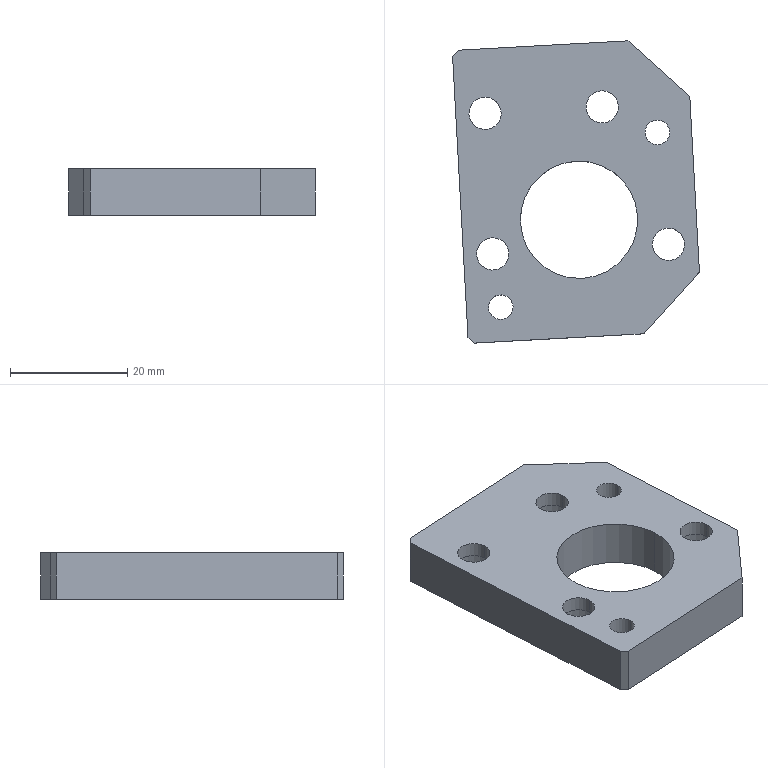Component | SolidWorks | T160418-M01U03-P13A-1 | 1 solid | 36 faces | box 42.07 x 51.51 x 8 mm | volume 10820 mm3 | cylinder 22 | plane 14 | commonest cylinder face diameters 9 x8 5.5 x8 4.2 x4 20 x2 | material S45C
STEP:
#1=COLOUR_RGB('',0.7922,0.8196,0.9333);
#2=FILL_AREA_STYLE_COLOUR('',#1);
#3=FILL_AREA_STYLE('',(#2));
#4=SURFACE_STYLE_FILL_AREA(#3);
#5=SURFACE_SIDE_STYLE('',(#4));
#6=SURFACE_STYLE_USAGE(.BOTH.,#5);
#7=PRESENTATION_STYLE_ASSIGNMENT((#6));
#8=CARTESIAN_POINT('',(19.336,6.191,-11.076));
#9=VERTEX_POINT('',#8);
#10=CARTESIAN_POINT('',(19.69,6.211,-11.076));
#11=VERTEX_POINT('',#10);
#12=CARTESIAN_POINT('',(19.513,6.201,-11.076));
#13=DIRECTION('',(0.,0.,-1.));
#14=DIRECTION('',(0.9985,0.05472,0.));
#15=AXIS2_PLACEMENT_3D('',#12,#13,#14);
#16=CIRCLE('',#15,0.1772);
#17=EDGE_CURVE('',#9,#11,#16,.T.);
#18=ORIENTED_EDGE('',*,*,#17,.F.);
#19=CARTESIAN_POINT('',(19.336,6.191,-11.292));
#20=VERTEX_POINT('',#19);
#21=CARTESIAN_POINT('',(19.336,6.191,-11.292));
#22=DIRECTION('',(0.,0.,-1.));
#23=VECTOR('',#22,39.37);
#24=LINE('',#21,#23);
#25=EDGE_CURVE('',#9,#20,#24,.T.);
#26=ORIENTED_EDGE('',*,*,#25,.T.);
#27=CARTESIAN_POINT('',(19.69,6.211,-11.292));
#28=VERTEX_POINT('',#27);
#29=CARTESIAN_POINT('',(19.513,6.201,-11.292));
#30=DIRECTION('',(0.,0.,-1.));
#31=DIRECTION('',(0.9985,0.05472,0.));
#32=AXIS2_PLACEMENT_3D('',#29,#30,#31);
#33=CIRCLE('',#32,0.1772);
#34=EDGE_CURVE('',#20,#28,#33,.T.);
#35=ORIENTED_EDGE('',*,*,#34,.T.);
#36=CARTESIAN_POINT('',(19.69,6.211,-11.292));
#37=DIRECTION('',(0.,0.,-1.));
#38=VECTOR('',#37,39.37);
#39=LINE('',#36,#38);
#40=EDGE_CURVE('',#11,#28,#39,.T.);
#41=ORIENTED_EDGE('',*,*,#40,.F.);
#42=EDGE_LOOP('',(#18,#26,#35,#41));
#43=FACE_OUTER_BOUND('',#42,.T.);
#44=CARTESIAN_POINT('',(19.513,6.201,-11.292));
#45=DIRECTION('',(0.,0.,-1.));
#46=DIRECTION('',(0.9985,0.05472,0.));
#47=AXIS2_PLACEMENT_3D('',#44,#45,#46);
#48=CYLINDRICAL_SURFACE('',#47,0.1772);
#49=ADVANCED_FACE('',(#43),#48,.F.);
#50=CARTESIAN_POINT('',(19.405,6.195,-10.977));
#51=VERTEX_POINT('',#50);
#52=CARTESIAN_POINT('',(19.621,6.207,-10.977));
#53=VERTEX_POINT('',#52);
#54=CARTESIAN_POINT('',(19.513,6.201,-10.977));
#55=DIRECTION('',(0.,0.,-1.));
#56=DIRECTION('',(0.9985,0.05472,0.));
#57=AXIS2_PLACEMENT_3D('',#54,#55,#56);
#58=CIRCLE('',#57,0.1083);
#59=EDGE_CURVE('',#51,#53,#58,.T.);
#60=ORIENTED_EDGE('',*,*,#59,.F.);
#61=CARTESIAN_POINT('',(19.405,6.195,-11.076));
#62=VERTEX_POINT('',#61);
#63=CARTESIAN_POINT('',(19.405,6.195,-11.292));
#64=DIRECTION('',(0.,0.,-1.));
#65=VECTOR('',#64,39.37);
#66=LINE('',#63,#65);
#67=EDGE_CURVE('',#51,#62,#66,.T.);
#68=ORIENTED_EDGE('',*,*,#67,.T.);
#69=CARTESIAN_POINT('',(19.621,6.207,-11.076));
#70=VERTEX_POINT('',#69);
#71=CARTESIAN_POINT('',(19.513,6.201,-11.076));
#72=DIRECTION('',(0.,0.,-1.));
#73=DIRECTION('',(0.9985,0.05472,0.));
#74=AXIS2_PLACEMENT_3D('',#71,#72,#73);
#75=CIRCLE('',#74,0.1083);
#76=EDGE_CURVE('',#62,#70,#75,.T.);
#77=ORIENTED_EDGE('',*,*,#76,.T.);
#78=CARTESIAN_POINT('',(19.621,6.207,-11.292));
#79=DIRECTION('',(0.,0.,-1.));
#80=VECTOR('',#79,39.37);
#81=LINE('',#78,#80);
#82=EDGE_CURVE('',#53,#70,#81,.T.);
#83=ORIENTED_EDGE('',*,*,#82,.F.);
#84=EDGE_LOOP('',(#60,#68,#77,#83));
#85=FACE_OUTER_BOUND('',#84,.T.);
#86=CARTESIAN_POINT('',(19.513,6.201,-11.292));
#87=DIRECTION('',(0.,0.,-1.));
#88=DIRECTION('',(0.9985,0.05472,0.));
#89=AXIS2_PLACEMENT_3D('',#86,#87,#88);
#90=CYLINDRICAL_SURFACE('',#89,0.1083);
#91=ADVANCED_FACE('',(#85),#90,.F.);
#92=CARTESIAN_POINT('',(19.388,5.248,-11.076));
#93=VERTEX_POINT('',#92);
#94=CARTESIAN_POINT('',(19.742,5.267,-11.076));
#95=VERTEX_POINT('',#94);
#96=CARTESIAN_POINT('',(19.565,5.257,-11.076));
#97=DIRECTION('',(0.,0.,-1.));
#98=DIRECTION('',(0.9985,0.05472,0.));
#99=AXIS2_PLACEMENT_3D('',#96,#97,#98);
#100=CIRCLE('',#99,0.1772);
#101=EDGE_CURVE('',#93,#95,#100,.T.);
#102=ORIENTED_EDGE('',*,*,#101,.F.);
#103=CARTESIAN_POINT('',(19.388,5.248,-11.292));
#104=VERTEX_POINT('',#103);
#105=CARTESIAN_POINT('',(19.388,5.248,-11.292));
#106=DIRECTION('',(0.,0.,-1.));
#107=VECTOR('',#106,39.37);
#108=LINE('',#105,#107);
#109=EDGE_CURVE('',#93,#104,#108,.T.);
#110=ORIENTED_EDGE('',*,*,#109,.T.);
#111=CARTESIAN_POINT('',(19.742,5.267,-11.292));
#112=VERTEX_POINT('',#111);
#113=CARTESIAN_POINT('',(19.565,5.257,-11.292));
#114=DIRECTION('',(0.,0.,-1.));
#115=DIRECTION('',(0.9985,0.05472,0.));
#116=AXIS2_PLACEMENT_3D('',#113,#114,#115);
#117=CIRCLE('',#116,0.1772);
#118=EDGE_CURVE('',#104,#112,#117,.T.);
#119=ORIENTED_EDGE('',*,*,#118,.T.);
#120=CARTESIAN_POINT('',(19.742,5.267,-11.292));
#121=DIRECTION('',(0.,0.,-1.));
#122=VECTOR('',#121,39.37);
#123=LINE('',#120,#122);
#124=EDGE_CURVE('',#95,#112,#123,.T.);
#125=ORIENTED_EDGE('',*,*,#124,.F.);
#126=EDGE_LOOP('',(#102,#110,#119,#125));
#127=FACE_OUTER_BOUND('',#126,.T.);
#128=CARTESIAN_POINT('',(19.565,5.257,-11.292));
#129=DIRECTION('',(0.,0.,-1.));
#130=DIRECTION('',(0.9985,0.05472,0.));
#131=AXIS2_PLACEMENT_3D('',#128,#129,#130);
#132=CYLINDRICAL_SURFACE('',#131,0.1772);
#133=ADVANCED_FACE('',(#127),#132,.F.);
#134=CARTESIAN_POINT('',(19.457,5.251,-10.977));
#135=VERTEX_POINT('',#134);
#136=CARTESIAN_POINT('',(19.673,5.263,-10.977));
#137=VERTEX_POINT('',#136);
#138=CARTESIAN_POINT('',(19.565,5.257,-10.977));
#139=DIRECTION('',(0.,0.,-1.));
#140=DIRECTION('',(0.9985,0.05472,0.));
#141=AXIS2_PLACEMENT_3D('',#138,#139,#140);
#142=CIRCLE('',#141,0.1083);
#143=EDGE_CURVE('',#135,#137,#142,.T.);
#144=ORIENTED_EDGE('',*,*,#143,.F.);
#145=CARTESIAN_POINT('',(19.457,5.251,-11.076));
#146=VERTEX_POINT('',#145);
#147=CARTESIAN_POINT('',(19.457,5.251,-11.292));
#148=DIRECTION('',(0.,0.,-1.));
#149=VECTOR('',#148,39.37);
#150=LINE('',#147,#149);
#151=EDGE_CURVE('',#135,#146,#150,.T.);
#152=ORIENTED_EDGE('',*,*,#151,.T.);
#153=CARTESIAN_POINT('',(19.673,5.263,-11.076));
#154=VERTEX_POINT('',#153);
#155=CARTESIAN_POINT('',(19.565,5.257,-11.076));
#156=DIRECTION('',(0.,0.,-1.));
#157=DIRECTION('',(0.9985,0.05472,0.));
#158=AXIS2_PLACEMENT_3D('',#155,#156,#157);
#159=CIRCLE('',#158,0.1083);
#160=EDGE_CURVE('',#146,#154,#159,.T.);
#161=ORIENTED_EDGE('',*,*,#160,.T.);
#162=CARTESIAN_POINT('',(19.673,5.263,-11.292));
#163=DIRECTION('',(0.,0.,-1.));
#164=VECTOR('',#163,39.37);
#165=LINE('',#162,#164);
#166=EDGE_CURVE('',#137,#154,#165,.T.);
#167=ORIENTED_EDGE('',*,*,#166,.F.);
#168=EDGE_LOOP('',(#144,#152,#161,#167));
#169=FACE_OUTER_BOUND('',#168,.T.);
#170=CARTESIAN_POINT('',(19.565,5.257,-11.292));
#171=DIRECTION('',(0.,0.,-1.));
#172=DIRECTION('',(0.9985,0.05472,0.));
#173=AXIS2_PLACEMENT_3D('',#170,#171,#172);
#174=CYLINDRICAL_SURFACE('',#173,0.1083);
#175=ADVANCED_FACE('',(#169),#174,.F.);
#176=CARTESIAN_POINT('',(20.122,6.234,-11.076));
#177=VERTEX_POINT('',#176);
#178=CARTESIAN_POINT('',(20.476,6.254,-11.076));
#179=VERTEX_POINT('',#178);
#180=CARTESIAN_POINT('',(20.299,6.244,-11.076));
#181=DIRECTION('',(0.,0.,-1.));
#182=DIRECTION('',(0.9985,0.05472,0.));
#183=AXIS2_PLACEMENT_3D('',#180,#181,#182);
#184=CIRCLE('',#183,0.1772);
#185=EDGE_CURVE('',#177,#179,#184,.T.);
#186=ORIENTED_EDGE('',*,*,#185,.F.);
#187=CARTESIAN_POINT('',(20.122,6.234,-11.292));
#188=VERTEX_POINT('',#187);
#189=CARTESIAN_POINT('',(20.122,6.234,-11.292));
#190=DIRECTION('',(0.,0.,-1.));
#191=VECTOR('',#190,39.37);
#192=LINE('',#189,#191);
#193=EDGE_CURVE('',#177,#188,#192,.T.);
#194=ORIENTED_EDGE('',*,*,#193,.T.);
#195=CARTESIAN_POINT('',(20.476,6.254,-11.292));
#196=VERTEX_POINT('',#195);
#197=CARTESIAN_POINT('',(20.299,6.244,-11.292));
#198=DIRECTION('',(0.,0.,-1.));
#199=DIRECTION('',(0.9985,0.05472,0.));
#200=AXIS2_PLACEMENT_3D('',#197,#198,#199);
#201=CIRCLE('',#200,0.1772);
#202=EDGE_CURVE('',#188,#196,#201,.T.);
#203=ORIENTED_EDGE('',*,*,#202,.T.);
#204=CARTESIAN_POINT('',(20.476,6.254,-11.292));
#205=DIRECTION('',(0.,0.,-1.));
#206=VECTOR('',#205,39.37);
#207=LINE('',#204,#206);
#208=EDGE_CURVE('',#179,#196,#207,.T.);
#209=ORIENTED_EDGE('',*,*,#208,.F.);
#210=EDGE_LOOP('',(#186,#194,#203,#209));
#211=FACE_OUTER_BOUND('',#210,.T.);
#212=CARTESIAN_POINT('',(20.299,6.244,-11.292));
#213=DIRECTION('',(0.,0.,-1.));
#214=DIRECTION('',(0.9985,0.05472,0.));
#215=AXIS2_PLACEMENT_3D('',#212,#213,#214);
#216=CYLINDRICAL_SURFACE('',#215,0.1772);
#217=ADVANCED_FACE('',(#211),#216,.F.);
#218=CARTESIAN_POINT('',(20.191,6.238,-10.977));
#219=VERTEX_POINT('',#218);
#220=CARTESIAN_POINT('',(20.407,6.25,-10.977));
#221=VERTEX_POINT('',#220);
#222=CARTESIAN_POINT('',(20.299,6.244,-10.977));
#223=DIRECTION('',(0.,0.,-1.));
#224=DIRECTION('',(0.9985,0.05472,0.));
#225=AXIS2_PLACEMENT_3D('',#222,#223,#224);
#226=CIRCLE('',#225,0.1083);
#227=EDGE_CURVE('',#219,#221,#226,.T.);
#228=ORIENTED_EDGE('',*,*,#227,.F.);
#229=CARTESIAN_POINT('',(20.191,6.238,-11.076));
#230=VERTEX_POINT('',#229);
#231=CARTESIAN_POINT('',(20.191,6.238,-11.292));
#232=DIRECTION('',(0.,0.,-1.));
#233=VECTOR('',#232,39.37);
#234=LINE('',#231,#233);
#235=EDGE_CURVE('',#219,#230,#234,.T.);
#236=ORIENTED_EDGE('',*,*,#235,.T.);
#237=CARTESIAN_POINT('',(20.407,6.25,-11.076));
#238=VERTEX_POINT('',#237);
#239=CARTESIAN_POINT('',(20.299,6.244,-11.076));
#240=DIRECTION('',(0.,0.,-1.));
#241=DIRECTION('',(0.9985,0.05472,0.));
#242=AXIS2_PLACEMENT_3D('',#239,#240,#241);
#243=CIRCLE('',#242,0.1083);
#244=EDGE_CURVE('',#230,#238,#243,.T.);
#245=ORIENTED_EDGE('',*,*,#244,.T.);
#246=CARTESIAN_POINT('',(20.407,6.25,-11.292));
#247=DIRECTION('',(0.,0.,-1.));
#248=VECTOR('',#247,39.37);
#249=LINE('',#246,#248);
#250=EDGE_CURVE('',#221,#238,#249,.T.);
#251=ORIENTED_EDGE('',*,*,#250,.F.);
#252=EDGE_LOOP('',(#228,#236,#245,#251));
#253=FACE_OUTER_BOUND('',#252,.T.);
#254=CARTESIAN_POINT('',(20.299,6.244,-11.292));
#255=DIRECTION('',(0.,0.,-1.));
#256=DIRECTION('',(0.9985,0.05472,0.));
#257=AXIS2_PLACEMENT_3D('',#254,#255,#256);
#258=CYLINDRICAL_SURFACE('',#257,0.1083);
#259=ADVANCED_FACE('',(#253),#258,.F.);
#260=CARTESIAN_POINT('',(20.567,5.312,-11.076));
#261=VERTEX_POINT('',#260);
#262=CARTESIAN_POINT('',(20.921,5.332,-11.076));
#263=VERTEX_POINT('',#262);
#264=CARTESIAN_POINT('',(20.744,5.322,-11.076));
#265=DIRECTION('',(0.,0.,-1.));
#266=DIRECTION('',(0.9985,0.05472,0.));
#267=AXIS2_PLACEMENT_3D('',#264,#265,#266);
#268=CIRCLE('',#267,0.1772);
#269=EDGE_CURVE('',#261,#263,#268,.T.);
#270=ORIENTED_EDGE('',*,*,#269,.F.);
#271=CARTESIAN_POINT('',(20.567,5.312,-11.292));
#272=VERTEX_POINT('',#271);
#273=CARTESIAN_POINT('',(20.567,5.312,-11.292));
#274=DIRECTION('',(0.,0.,-1.));
#275=VECTOR('',#274,39.37);
#276=LINE('',#273,#275);
#277=EDGE_CURVE('',#261,#272,#276,.T.);
#278=ORIENTED_EDGE('',*,*,#277,.T.);
#279=CARTESIAN_POINT('',(20.921,5.332,-11.292));
#280=VERTEX_POINT('',#279);
#281=CARTESIAN_POINT('',(20.744,5.322,-11.292));
#282=DIRECTION('',(0.,0.,-1.));
#283=DIRECTION('',(0.9985,0.05472,0.));
#284=AXIS2_PLACEMENT_3D('',#281,#282,#283);
#285=CIRCLE('',#284,0.1772);
#286=EDGE_CURVE('',#272,#280,#285,.T.);
#287=ORIENTED_EDGE('',*,*,#286,.T.);
#288=CARTESIAN_POINT('',(20.921,5.332,-11.292));
#289=DIRECTION('',(0.,0.,-1.));
#290=VECTOR('',#289,39.37);
#291=LINE('',#288,#290);
#292=EDGE_CURVE('',#263,#280,#291,.T.);
#293=ORIENTED_EDGE('',*,*,#292,.F.);
#294=EDGE_LOOP('',(#270,#278,#287,#293));
#295=FACE_OUTER_BOUND('',#294,.T.);
#296=CARTESIAN_POINT('',(20.744,5.322,-11.292));
#297=DIRECTION('',(0.,0.,-1.));
#298=DIRECTION('',(0.9985,0.05472,0.));
#299=AXIS2_PLACEMENT_3D('',#296,#297,#298);
#300=CYLINDRICAL_SURFACE('',#299,0.1772);
#301=ADVANCED_FACE('',(#295),#300,.F.);
#302=CARTESIAN_POINT('',(20.636,5.316,-10.977));
#303=VERTEX_POINT('',#302);
#304=CARTESIAN_POINT('',(20.852,5.328,-10.977));
#305=VERTEX_POINT('',#304);
#306=CARTESIAN_POINT('',(20.744,5.322,-10.977));
#307=DIRECTION('',(0.,0.,-1.));
#308=DIRECTION('',(0.9985,0.05472,0.));
#309=AXIS2_PLACEMENT_3D('',#306,#307,#308);
#310=CIRCLE('',#309,0.1083);
#311=EDGE_CURVE('',#303,#305,#310,.T.);
#312=ORIENTED_EDGE('',*,*,#311,.F.);
#313=CARTESIAN_POINT('',(20.636,5.316,-11.076));
#314=VERTEX_POINT('',#313);
#315=CARTESIAN_POINT('',(20.636,5.316,-11.292));
#316=DIRECTION('',(0.,0.,-1.));
#317=VECTOR('',#316,39.37);
#318=LINE('',#315,#317);
#319=EDGE_CURVE('',#303,#314,#318,.T.);
#320=ORIENTED_EDGE('',*,*,#319,.T.);
#321=CARTESIAN_POINT('',(20.852,5.328,-11.076));
#322=VERTEX_POINT('',#321);
#323=CARTESIAN_POINT('',(20.744,5.322,-11.076));
#324=DIRECTION('',(0.,0.,-1.));
#325=DIRECTION('',(0.9985,0.05472,0.));
#326=AXIS2_PLACEMENT_3D('',#323,#324,#325);
#327=CIRCLE('',#326,0.1083);
#328=EDGE_CURVE('',#314,#322,#327,.T.);
#329=ORIENTED_EDGE('',*,*,#328,.T.);
#330=CARTESIAN_POINT('',(20.852,5.328,-11.292));
#331=DIRECTION('',(0.,0.,-1.));
#332=VECTOR('',#331,39.37);
#333=LINE('',#330,#332);
#334=EDGE_CURVE('',#305,#322,#333,.T.);
#335=ORIENTED_EDGE('',*,*,#334,.F.);
#336=EDGE_LOOP('',(#312,#320,#329,#335));
#337=FACE_OUTER_BOUND('',#336,.T.);
#338=CARTESIAN_POINT('',(20.744,5.322,-11.292));
#339=DIRECTION('',(0.,0.,-1.));
#340=DIRECTION('',(0.9985,0.05472,0.));
#341=AXIS2_PLACEMENT_3D('',#338,#339,#340);
#342=CYLINDRICAL_SURFACE('',#341,0.1083);
#343=ADVANCED_FACE('',(#337),#342,.F.);
#344=CARTESIAN_POINT('',(20.587,6.068,-10.977));
#345=VERTEX_POINT('',#344);
#346=CARTESIAN_POINT('',(20.752,6.078,-10.977));
#347=VERTEX_POINT('',#346);
#348=CARTESIAN_POINT('',(20.669,6.073,-10.977));
#349=DIRECTION('',(0.,0.,-1.));
#350=DIRECTION('',(0.9985,0.05472,0.));
#351=AXIS2_PLACEMENT_3D('',#348,#349,#350);
#352=CIRCLE('',#351,0.08268);
#353=EDGE_CURVE('',#345,#347,#352,.T.);
#354=ORIENTED_EDGE('',*,*,#353,.F.);
#355=CARTESIAN_POINT('',(20.587,6.068,-11.292));
#356=VERTEX_POINT('',#355);
#357=CARTESIAN_POINT('',(20.587,6.068,-11.292));
#358=DIRECTION('',(0.,0.,-1.));
#359=VECTOR('',#358,39.37);
#360=LINE('',#357,#359);
#361=EDGE_CURVE('',#345,#356,#360,.T.);
#362=ORIENTED_EDGE('',*,*,#361,.T.);
#363=CARTESIAN_POINT('',(20.752,6.078,-11.292));
#364=VERTEX_POINT('',#363);
#365=CARTESIAN_POINT('',(20.669,6.073,-11.292));
#366=DIRECTION('',(0.,0.,-1.));
#367=DIRECTION('',(0.9985,0.05472,0.));
#368=AXIS2_PLACEMENT_3D('',#365,#366,#367);
#369=CIRCLE('',#368,0.08268);
#370=EDGE_CURVE('',#356,#364,#369,.T.);
#371=ORIENTED_EDGE('',*,*,#370,.T.);
#372=CARTESIAN_POINT('',(20.752,6.078,-11.292));
#373=DIRECTION('',(0.,0.,-1.));
#374=VECTOR('',#373,39.37);
#375=LINE('',#372,#374);
#376=EDGE_CURVE('',#347,#364,#375,.T.);
#377=ORIENTED_EDGE('',*,*,#376,.F.);
#378=EDGE_LOOP('',(#354,#362,#371,#377));
#379=FACE_OUTER_BOUND('',#378,.T.);
#380=CARTESIAN_POINT('',(20.669,6.073,-11.292));
#381=DIRECTION('',(0.,0.,-1.));
#382=DIRECTION('',(0.9985,0.05472,0.));
#383=AXIS2_PLACEMENT_3D('',#380,#381,#382);
#384=CYLINDRICAL_SURFACE('',#383,0.08268);
#385=ADVANCED_FACE('',(#379),#384,.F.);
#386=CARTESIAN_POINT('',(19.536,4.895,-10.977));
#387=VERTEX_POINT('',#386);
#388=CARTESIAN_POINT('',(19.701,4.904,-10.977));
#389=VERTEX_POINT('',#388);
#390=CARTESIAN_POINT('',(19.618,4.9,-10.977));
#391=DIRECTION('',(0.,0.,-1.));
#392=DIRECTION('',(0.9985,0.05472,0.));
#393=AXIS2_PLACEMENT_3D('',#390,#391,#392);
#394=CIRCLE('',#393,0.08268);
#395=EDGE_CURVE('',#387,#389,#394,.T.);
#396=ORIENTED_EDGE('',*,*,#395,.F.);
#397=CARTESIAN_POINT('',(19.536,4.895,-11.292));
#398=VERTEX_POINT('',#397);
#399=CARTESIAN_POINT('',(19.536,4.895,-11.292));
#400=DIRECTION('',(0.,0.,-1.));
#401=VECTOR('',#400,39.37);
#402=LINE('',#399,#401);
#403=EDGE_CURVE('',#387,#398,#402,.T.);
#404=ORIENTED_EDGE('',*,*,#403,.T.);
#405=CARTESIAN_POINT('',(19.701,4.904,-11.292));
#406=VERTEX_POINT('',#405);
#407=CARTESIAN_POINT('',(19.618,4.9,-11.292));
#408=DIRECTION('',(0.,0.,-1.));
#409=DIRECTION('',(0.9985,0.05472,0.));
#410=AXIS2_PLACEMENT_3D('',#407,#408,#409);
#411=CIRCLE('',#410,0.08268);
#412=EDGE_CURVE('',#398,#406,#411,.T.);
#413=ORIENTED_EDGE('',*,*,#412,.T.);
#414=CARTESIAN_POINT('',(19.701,4.904,-11.292));
#415=DIRECTION('',(0.,0.,-1.));
#416=VECTOR('',#415,39.37);
#417=LINE('',#414,#416);
#418=EDGE_CURVE('',#389,#406,#417,.T.);
#419=ORIENTED_EDGE('',*,*,#418,.F.);
#420=EDGE_LOOP('',(#396,#404,#413,#419));
#421=FACE_OUTER_BOUND('',#420,.T.);
#422=CARTESIAN_POINT('',(19.618,4.9,-11.292));
#423=DIRECTION('',(0.,0.,-1.));
#424=DIRECTION('',(0.9985,0.05472,0.));
#425=AXIS2_PLACEMENT_3D('',#422,#423,#424);
#426=CYLINDRICAL_SURFACE('',#425,0.08268);
#427=ADVANCED_FACE('',(#421),#426,.F.);
#428=CARTESIAN_POINT('',(20.537,5.508,-10.977));
#429=VERTEX_POINT('',#428);
#430=CARTESIAN_POINT('',(19.751,5.465,-10.977));
#431=VERTEX_POINT('',#430);
#432=CARTESIAN_POINT('',(20.144,5.486,-10.977));
#433=DIRECTION('',(-0.,-0.,1.));
#434=DIRECTION('',(-0.9985,-0.05472,0.));
#435=AXIS2_PLACEMENT_3D('',#432,#433,#434);
#436=CIRCLE('',#435,0.3937);
#437=EDGE_CURVE('',#429,#431,#436,.T.);
#438=ORIENTED_EDGE('',*,*,#437,.T.);
#439=CARTESIAN_POINT('',(19.751,5.465,-11.292));
#440=VERTEX_POINT('',#439);
#441=CARTESIAN_POINT('',(19.751,5.465,-10.977));
#442=DIRECTION('',(0.,0.,-1.));
#443=VECTOR('',#442,39.37);
#444=LINE('',#441,#443);
#445=EDGE_CURVE('',#431,#440,#444,.T.);
#446=ORIENTED_EDGE('',*,*,#445,.T.);
#447=CARTESIAN_POINT('',(20.537,5.508,-11.292));
#448=VERTEX_POINT('',#447);
#449=CARTESIAN_POINT('',(20.144,5.486,-11.292));
#450=DIRECTION('',(-0.,-0.,1.));
#451=DIRECTION('',(-0.9985,-0.05472,0.));
#452=AXIS2_PLACEMENT_3D('',#449,#450,#451);
#453=CIRCLE('',#452,0.3937);
#454=EDGE_CURVE('',#448,#440,#453,.T.);
#455=ORIENTED_EDGE('',*,*,#454,.F.);
#456=CARTESIAN_POINT('',(20.537,5.508,-10.977));
#457=DIRECTION('',(0.,0.,-1.));
#458=VECTOR('',#457,39.37);
#459=LINE('',#456,#458);
#460=EDGE_CURVE('',#429,#448,#459,.T.);
#461=ORIENTED_EDGE('',*,*,#460,.F.);
#462=EDGE_LOOP('',(#438,#446,#455,#461));
#463=FACE_OUTER_BOUND('',#462,.T.);
#464=CARTESIAN_POINT('',(20.144,5.486,-10.977));
#465=DIRECTION('',(0.,0.,-1.));
#466=DIRECTION('',(0.9985,0.05472,0.));
#467=AXIS2_PLACEMENT_3D('',#464,#465,#466);
#468=CYLINDRICAL_SURFACE('',#467,0.3937);
#469=ADVANCED_FACE('',(#463),#468,.F.);
#470=CARTESIAN_POINT('',(19.513,6.201,-11.292));
#471=DIRECTION('',(0.,0.,-1.));
#472=DIRECTION('',(0.9985,0.05472,0.));
#473=AXIS2_PLACEMENT_3D('',#470,#471,#472);
#474=CIRCLE('',#473,0.1772);
#475=EDGE_CURVE('',#28,#20,#474,.T.);
#476=ORIENTED_EDGE('',*,*,#475,.F.);
#477=ORIENTED_EDGE('',*,*,#34,.F.);
#478=EDGE_LOOP('',(#476,#477));
#479=FACE_BOUND('',#478,.T.);
#480=CARTESIAN_POINT('',(19.565,5.257,-11.292));
#481=DIRECTION('',(0.,0.,-1.));
#482=DIRECTION('',(0.9985,0.05472,0.));
#483=AXIS2_PLACEMENT_3D('',#480,#481,#482);
#484=CIRCLE('',#483,0.1772);
#485=EDGE_CURVE('',#112,#104,#484,.T.);
#486=ORIENTED_EDGE('',*,*,#485,.F.);
#487=ORIENTED_EDGE('',*,*,#118,.F.);
#488=EDGE_LOOP('',(#486,#487));
#489=FACE_BOUND('',#488,.T.);
#490=CARTESIAN_POINT('',(20.299,6.244,-11.292));
#491=DIRECTION('',(0.,0.,-1.));
#492=DIRECTION('',(0.9985,0.05472,0.));
#493=AXIS2_PLACEMENT_3D('',#490,#491,#492);
#494=CIRCLE('',#493,0.1772);
#495=EDGE_CURVE('',#196,#188,#494,.T.);
#496=ORIENTED_EDGE('',*,*,#495,.F.);
#497=ORIENTED_EDGE('',*,*,#202,.F.);
#498=EDGE_LOOP('',(#496,#497));
#499=FACE_BOUND('',#498,.T.);
#500=CARTESIAN_POINT('',(20.744,5.322,-11.292));
#501=DIRECTION('',(0.,0.,-1.));
#502=DIRECTION('',(0.9985,0.05472,0.));
#503=AXIS2_PLACEMENT_3D('',#500,#501,#502);
#504=CIRCLE('',#503,0.1772);
#505=EDGE_CURVE('',#280,#272,#504,.T.);
#506=ORIENTED_EDGE('',*,*,#505,.F.);
#507=ORIENTED_EDGE('',*,*,#286,.F.);
#508=EDGE_LOOP('',(#506,#507));
#509=FACE_BOUND('',#508,.T.);
#510=CARTESIAN_POINT('',(20.669,6.073,-11.292));
#511=DIRECTION('',(0.,0.,-1.));
#512=DIRECTION('',(0.9985,0.05472,0.));
#513=AXIS2_PLACEMENT_3D('',#510,#511,#512);
#514=CIRCLE('',#513,0.08268);
#515=EDGE_CURVE('',#364,#356,#514,.T.);
#516=ORIENTED_EDGE('',*,*,#515,.F.);
#517=ORIENTED_EDGE('',*,*,#370,.F.);
#518=EDGE_LOOP('',(#516,#517));
#519=FACE_BOUND('',#518,.T.);
#520=CARTESIAN_POINT('',(19.44,4.659,-11.292));
#521=VERTEX_POINT('',#520);
#522=CARTESIAN_POINT('',(20.58,4.722,-11.292));
#523=VERTEX_POINT('',#522);
#524=CARTESIAN_POINT('',(20.973,4.743,-11.292));
#525=DIRECTION('',(0.9985,0.05472,0.));
#526=VECTOR('',#525,39.37);
#527=LINE('',#524,#526);
#528=EDGE_CURVE('',#521,#523,#527,.T.);
#529=ORIENTED_EDGE('',*,*,#528,.F.);
#530=CARTESIAN_POINT('',(19.398,4.696,-11.292));
#531=VERTEX_POINT('',#530);
#532=CARTESIAN_POINT('',(19.44,4.659,-11.292));
#533=DIRECTION('',(-0.7447,0.6674,-0.));
#534=VECTOR('',#533,39.37);
#535=LINE('',#532,#534);
#536=EDGE_CURVE('',#521,#531,#535,.T.);
#537=ORIENTED_EDGE('',*,*,#536,.T.);
#538=CARTESIAN_POINT('',(19.295,6.583,-11.292));
#539=VERTEX_POINT('',#538);
#540=CARTESIAN_POINT('',(19.401,4.657,-11.292));
#541=DIRECTION('',(0.05472,-0.9985,-0.));
#542=VECTOR('',#541,39.37);
#543=LINE('',#540,#542);
#544=EDGE_CURVE('',#539,#531,#543,.T.);
#545=ORIENTED_EDGE('',*,*,#544,.F.);
#546=CARTESIAN_POINT('',(19.332,6.625,-11.292));
#547=VERTEX_POINT('',#546);
#548=CARTESIAN_POINT('',(19.295,6.583,-11.292));
#549=DIRECTION('',(0.6674,0.7447,0.));
#550=VECTOR('',#549,39.37);
#551=LINE('',#548,#550);
#552=EDGE_CURVE('',#539,#547,#551,.T.);
#553=ORIENTED_EDGE('',*,*,#552,.T.);
#554=CARTESIAN_POINT('',(20.472,6.687,-11.292));
#555=VERTEX_POINT('',#554);
#556=CARTESIAN_POINT('',(20.865,6.709,-11.292));
#557=DIRECTION('',(-0.9985,-0.05472,-0.));
#558=VECTOR('',#557,39.37);
#559=LINE('',#556,#558);
#560=EDGE_CURVE('',#555,#547,#559,.T.);
#561=ORIENTED_EDGE('',*,*,#560,.F.);
#562=CARTESIAN_POINT('',(20.887,6.316,-11.292));
#563=VERTEX_POINT('',#562);
#564=CARTESIAN_POINT('',(20.472,6.687,-11.292));
#565=DIRECTION('',(0.7447,-0.6674,0.));
#566=VECTOR('',#565,39.37);
#567=LINE('',#564,#566);
#568=EDGE_CURVE('',#555,#563,#567,.T.);
#569=ORIENTED_EDGE('',*,*,#568,.T.);
#570=CARTESIAN_POINT('',(20.951,5.136,-11.292));
#571=VERTEX_POINT('',#570);
#572=CARTESIAN_POINT('',(20.973,4.743,-11.292));
#573=DIRECTION('',(-0.05472,0.9985,0.));
#574=VECTOR('',#573,39.37);
#575=LINE('',#572,#574);
#576=EDGE_CURVE('',#571,#563,#575,.T.);
#577=ORIENTED_EDGE('',*,*,#576,.F.);
#578=CARTESIAN_POINT('',(20.951,5.136,-11.292));
#579=DIRECTION('',(-0.6674,-0.7447,-0.));
#580=VECTOR('',#579,39.37);
#581=LINE('',#578,#580);
#582=EDGE_CURVE('',#571,#523,#581,.T.);
#583=ORIENTED_EDGE('',*,*,#582,.T.);
#584=EDGE_LOOP('',(#529,#537,#545,#553,#561,#569,#577,#583));
#585=FACE_OUTER_BOUND('',#584,.T.);
#586=ORIENTED_EDGE('',*,*,#454,.T.);
#587=CARTESIAN_POINT('',(20.144,5.486,-11.292));
#588=DIRECTION('',(-0.,-0.,1.));
#589=DIRECTION('',(-0.9985,-0.05472,0.));
#590=AXIS2_PLACEMENT_3D('',#587,#588,#589);
#591=CIRCLE('',#590,0.3937);
#592=EDGE_CURVE('',#440,#448,#591,.T.);
#593=ORIENTED_EDGE('',*,*,#592,.T.);
#594=EDGE_LOOP('',(#586,#593));
#595=FACE_BOUND('',#594,.T.);
#596=CARTESIAN_POINT('',(19.618,4.9,-11.292));
#597=DIRECTION('',(0.,0.,-1.));
#598=DIRECTION('',(0.9985,0.05472,0.));
#599=AXIS2_PLACEMENT_3D('',#596,#597,#598);
#600=CIRCLE('',#599,0.08268);
#601=EDGE_CURVE('',#406,#398,#600,.T.);
#602=ORIENTED_EDGE('',*,*,#601,.F.);
#603=ORIENTED_EDGE('',*,*,#412,.F.);
#604=EDGE_LOOP('',(#602,#603));
#605=FACE_BOUND('',#604,.T.);
#606=CARTESIAN_POINT('',(19.293,6.623,-11.292));
#607=DIRECTION('',(-0.,-0.,1.));
#608=DIRECTION('',(-0.9985,-0.05472,-0.));
#609=AXIS2_PLACEMENT_3D('',#606,#607,#608);
#610=PLANE('',#609);
#611=ADVANCED_FACE('',(#479,#489,#499,#509,#519,#585,#595,#605),#610,.F.);
#612=CARTESIAN_POINT('',(19.513,6.201,-10.977));
#613=DIRECTION('',(0.,0.,-1.));
#614=DIRECTION('',(0.9985,0.05472,0.));
#615=AXIS2_PLACEMENT_3D('',#612,#613,#614);
#616=CIRCLE('',#615,0.1083);
#617=EDGE_CURVE('',#53,#51,#616,.T.);
#618=ORIENTED_EDGE('',*,*,#617,.T.);
#619=ORIENTED_EDGE('',*,*,#59,.T.);
#620=EDGE_LOOP('',(#618,#619));
#621=FACE_BOUND('',#620,.T.);
#622=CARTESIAN_POINT('',(19.565,5.257,-10.977));
#623=DIRECTION('',(0.,0.,-1.));
#624=DIRECTION('',(0.9985,0.05472,0.));
#625=AXIS2_PLACEMENT_3D('',#622,#623,#624);
#626=CIRCLE('',#625,0.1083);
#627=EDGE_CURVE('',#137,#135,#626,.T.);
#628=ORIENTED_EDGE('',*,*,#627,.T.);
#629=ORIENTED_EDGE('',*,*,#143,.T.);
#630=EDGE_LOOP('',(#628,#629));
#631=FACE_BOUND('',#630,.T.);
#632=CARTESIAN_POINT('',(20.299,6.244,-10.977));
#633=DIRECTION('',(0.,0.,-1.));
#634=DIRECTION('',(0.9985,0.05472,0.));
#635=AXIS2_PLACEMENT_3D('',#632,#633,#634);
#636=CIRCLE('',#635,0.1083);
#637=EDGE_CURVE('',#221,#219,#636,.T.);
#638=ORIENTED_EDGE('',*,*,#637,.T.);
#639=ORIENTED_EDGE('',*,*,#227,.T.);
#640=EDGE_LOOP('',(#638,#639));
#641=FACE_BOUND('',#640,.T.);
#642=CARTESIAN_POINT('',(20.744,5.322,-10.977));
#643=DIRECTION('',(0.,0.,-1.));
#644=DIRECTION('',(0.9985,0.05472,0.));
#645=AXIS2_PLACEMENT_3D('',#642,#643,#644);
#646=CIRCLE('',#645,0.1083);
#647=EDGE_CURVE('',#305,#303,#646,.T.);
#648=ORIENTED_EDGE('',*,*,#647,.T.);
#649=ORIENTED_EDGE('',*,*,#311,.T.);
#650=EDGE_LOOP('',(#648,#649));
#651=FACE_BOUND('',#650,.T.);
#652=CARTESIAN_POINT('',(20.669,6.073,-10.977));
#653=DIRECTION('',(0.,0.,-1.));
#654=DIRECTION('',(0.9985,0.05472,0.));
#655=AXIS2_PLACEMENT_3D('',#652,#653,#654);
#656=CIRCLE('',#655,0.08268);
#657=EDGE_CURVE('',#347,#345,#656,.T.);
#658=ORIENTED_EDGE('',*,*,#657,.T.);
#659=ORIENTED_EDGE('',*,*,#353,.T.);
#660=EDGE_LOOP('',(#658,#659));
#661=FACE_BOUND('',#660,.T.);
#662=CARTESIAN_POINT('',(19.618,4.9,-10.977));
#663=DIRECTION('',(0.,0.,-1.));
#664=DIRECTION('',(0.9985,0.05472,0.));
#665=AXIS2_PLACEMENT_3D('',#662,#663,#664);
#666=CIRCLE('',#665,0.08268);
#667=EDGE_CURVE('',#389,#387,#666,.T.);
#668=ORIENTED_EDGE('',*,*,#667,.T.);
#669=ORIENTED_EDGE('',*,*,#395,.T.);
#670=EDGE_LOOP('',(#668,#669));
#671=FACE_BOUND('',#670,.T.);
#672=CARTESIAN_POINT('',(19.295,6.583,-10.977));
#673=VERTEX_POINT('',#672);
#674=CARTESIAN_POINT('',(19.398,4.696,-10.977));
#675=VERTEX_POINT('',#674);
#676=CARTESIAN_POINT('',(19.401,4.657,-10.977));
#677=DIRECTION('',(0.05472,-0.9985,-0.));
#678=VECTOR('',#677,39.37);
#679=LINE('',#676,#678);
#680=EDGE_CURVE('',#673,#675,#679,.T.);
#681=ORIENTED_EDGE('',*,*,#680,.T.);
#682=CARTESIAN_POINT('',(19.44,4.659,-10.977));
#683=VERTEX_POINT('',#682);
#684=CARTESIAN_POINT('',(18.382,5.607,-10.977));
#685=DIRECTION('',(0.7447,-0.6674,0.));
#686=VECTOR('',#685,39.37);
#687=LINE('',#684,#686);
#688=EDGE_CURVE('',#675,#683,#687,.T.);
#689=ORIENTED_EDGE('',*,*,#688,.T.);
#690=CARTESIAN_POINT('',(20.58,4.722,-10.977));
#691=VERTEX_POINT('',#690);
#692=CARTESIAN_POINT('',(20.973,4.743,-10.977));
#693=DIRECTION('',(0.9985,0.05472,0.));
#694=VECTOR('',#693,39.37);
#695=LINE('',#692,#694);
#696=EDGE_CURVE('',#683,#691,#695,.T.);
#697=ORIENTED_EDGE('',*,*,#696,.T.);
#698=CARTESIAN_POINT('',(20.951,5.136,-10.977));
#699=VERTEX_POINT('',#698);
#700=CARTESIAN_POINT('',(20.951,5.136,-10.977));
#701=DIRECTION('',(0.6674,0.7447,0.));
#702=VECTOR('',#701,39.37);
#703=LINE('',#700,#702);
#704=EDGE_CURVE('',#691,#699,#703,.T.);
#705=ORIENTED_EDGE('',*,*,#704,.T.);
#706=CARTESIAN_POINT('',(20.887,6.316,-10.977));
#707=VERTEX_POINT('',#706);
#708=CARTESIAN_POINT('',(20.973,4.743,-10.977));
#709=DIRECTION('',(-0.05472,0.9985,0.));
#710=VECTOR('',#709,39.37);
#711=LINE('',#708,#710);
#712=EDGE_CURVE('',#699,#707,#711,.T.);
#713=ORIENTED_EDGE('',*,*,#712,.T.);
#714=CARTESIAN_POINT('',(20.472,6.687,-10.977));
#715=VERTEX_POINT('',#714);
#716=CARTESIAN_POINT('',(19.85,7.244,-10.977));
#717=DIRECTION('',(-0.7447,0.6674,-0.));
#718=VECTOR('',#717,39.37);
#719=LINE('',#716,#718);
#720=EDGE_CURVE('',#707,#715,#719,.T.);
#721=ORIENTED_EDGE('',*,*,#720,.T.);
#722=CARTESIAN_POINT('',(19.332,6.625,-10.977));
#723=VERTEX_POINT('',#722);
#724=CARTESIAN_POINT('',(20.865,6.709,-10.977));
#725=DIRECTION('',(-0.9985,-0.05472,-0.));
#726=VECTOR('',#725,39.37);
#727=LINE('',#724,#726);
#728=EDGE_CURVE('',#715,#723,#727,.T.);
#729=ORIENTED_EDGE('',*,*,#728,.T.);
#730=CARTESIAN_POINT('',(19.314,6.604,-10.977));
#731=DIRECTION('',(-0.6674,-0.7447,-0.));
#732=VECTOR('',#731,39.37);
#733=LINE('',#730,#732);
#734=EDGE_CURVE('',#723,#673,#733,.T.);
#735=ORIENTED_EDGE('',*,*,#734,.T.);
#736=EDGE_LOOP('',(#681,#689,#697,#705,#713,#721,#729,#735));
#737=FACE_OUTER_BOUND('',#736,.T.);
#738=ORIENTED_EDGE('',*,*,#437,.F.);
#739=CARTESIAN_POINT('',(20.144,5.486,-10.977));
#740=DIRECTION('',(-0.,-0.,1.));
#741=DIRECTION('',(-0.9985,-0.05472,0.));
#742=AXIS2_PLACEMENT_3D('',#739,#740,#741);
#743=CIRCLE('',#742,0.3937);
#744=EDGE_CURVE('',#431,#429,#743,.T.);
#745=ORIENTED_EDGE('',*,*,#744,.F.);
#746=EDGE_LOOP('',(#738,#745));
#747=FACE_BOUND('',#746,.T.);
#748=CARTESIAN_POINT('',(19.293,6.623,-10.977));
#749=DIRECTION('',(-0.,-0.,1.));
#750=DIRECTION('',(-0.9985,-0.05472,-0.));
#751=AXIS2_PLACEMENT_3D('',#748,#749,#750);
#752=PLANE('',#751);
#753=ADVANCED_FACE('',(#621,#631,#641,#651,#661,#671,#737,#747),#752,.T.);
#754=ORIENTED_EDGE('',*,*,#544,.T.);
#755=CARTESIAN_POINT('',(19.398,4.696,-10.977));
#756=DIRECTION('',(-0.,-0.,1.));
#757=VECTOR('',#756,39.37);
#758=LINE('',#755,#757);
#759=EDGE_CURVE('',#531,#675,#758,.T.);
#760=ORIENTED_EDGE('',*,*,#759,.T.);
#761=ORIENTED_EDGE('',*,*,#680,.F.);
#762=CARTESIAN_POINT('',(19.295,6.583,-10.977));
#763=DIRECTION('',(0.,0.,-1.));
#764=VECTOR('',#763,39.37);
#765=LINE('',#762,#764);
#766=EDGE_CURVE('',#673,#539,#765,.T.);
#767=ORIENTED_EDGE('',*,*,#766,.T.);
#768=EDGE_LOOP('',(#754,#760,#761,#767));
#769=FACE_OUTER_BOUND('',#768,.T.);
#770=CARTESIAN_POINT('',(19.401,4.657,-10.977));
#771=DIRECTION('',(0.9985,0.05472,0.));
#772=DIRECTION('',(-0.,-0.,1.));
#773=AXIS2_PLACEMENT_3D('',#770,#771,#772);
#774=PLANE('',#773);
#775=ADVANCED_FACE('',(#769),#774,.F.);
#776=ORIENTED_EDGE('',*,*,#696,.F.);
#777=CARTESIAN_POINT('',(19.44,4.659,-10.977));
#778=DIRECTION('',(0.,0.,-1.));
#779=VECTOR('',#778,39.37);
#780=LINE('',#777,#779);
#781=EDGE_CURVE('',#683,#521,#780,.T.);
#782=ORIENTED_EDGE('',*,*,#781,.T.);
#783=ORIENTED_EDGE('',*,*,#528,.T.);
#784=CARTESIAN_POINT('',(20.58,4.722,-10.977));
#785=DIRECTION('',(-0.,-0.,1.));
#786=VECTOR('',#785,39.37);
#787=LINE('',#784,#786);
#788=EDGE_CURVE('',#523,#691,#787,.T.);
#789=ORIENTED_EDGE('',*,*,#788,.T.);
#790=EDGE_LOOP('',(#776,#782,#783,#789));
#791=FACE_OUTER_BOUND('',#790,.T.);
#792=CARTESIAN_POINT('',(20.973,4.743,-10.977));
#793=DIRECTION('',(-0.05472,0.9985,0.));
#794=DIRECTION('',(0.,0.,-1.));
#795=AXIS2_PLACEMENT_3D('',#792,#793,#794);
#796=PLANE('',#795);
#797=ADVANCED_FACE('',(#791),#796,.F.);
#798=ORIENTED_EDGE('',*,*,#576,.T.);
#799=CARTESIAN_POINT('',(20.887,6.316,-10.977));
#800=DIRECTION('',(-0.,-0.,1.));
#801=VECTOR('',#800,39.37);
#802=LINE('',#799,#801);
#803=EDGE_CURVE('',#563,#707,#802,.T.);
#804=ORIENTED_EDGE('',*,*,#803,.T.);
#805=ORIENTED_EDGE('',*,*,#712,.F.);
#806=CARTESIAN_POINT('',(20.951,5.136,-10.977));
#807=DIRECTION('',(0.,0.,-1.));
#808=VECTOR('',#807,39.37);
#809=LINE('',#806,#808);
#810=EDGE_CURVE('',#699,#571,#809,.T.);
#811=ORIENTED_EDGE('',*,*,#810,.T.);
#812=EDGE_LOOP('',(#798,#804,#805,#811));
#813=FACE_OUTER_BOUND('',#812,.T.);
#814=CARTESIAN_POINT('',(20.973,4.743,-10.977));
#815=DIRECTION('',(-0.9985,-0.05472,-0.));
#816=DIRECTION('',(0.05472,-0.9985,-0.));
#817=AXIS2_PLACEMENT_3D('',#814,#815,#816);
#818=PLANE('',#817);
#819=ADVANCED_FACE('',(#813),#818,.F.);
#820=ORIENTED_EDGE('',*,*,#560,.T.);
#821=CARTESIAN_POINT('',(19.332,6.625,-10.977));
#822=DIRECTION('',(-0.,-0.,1.));
#823=VECTOR('',#822,39.37);
#824=LINE('',#821,#823);
#825=EDGE_CURVE('',#547,#723,#824,.T.);
#826=ORIENTED_EDGE('',*,*,#825,.T.);
#827=ORIENTED_EDGE('',*,*,#728,.F.);
#828=CARTESIAN_POINT('',(20.472,6.687,-10.977));
#829=DIRECTION('',(0.,0.,-1.));
#830=VECTOR('',#829,39.37);
#831=LINE('',#828,#830);
#832=EDGE_CURVE('',#715,#555,#831,.T.);
#833=ORIENTED_EDGE('',*,*,#832,.T.);
#834=EDGE_LOOP('',(#820,#826,#827,#833));
#835=FACE_OUTER_BOUND('',#834,.T.);
#836=CARTESIAN_POINT('',(20.865,6.709,-10.977));
#837=DIRECTION('',(0.05472,-0.9985,-0.));
#838=DIRECTION('',(-0.,-0.,1.));
#839=AXIS2_PLACEMENT_3D('',#836,#837,#838);
#840=PLANE('',#839);
#841=ADVANCED_FACE('',(#835),#840,.F.);
#842=ORIENTED_EDGE('',*,*,#445,.F.);
#843=ORIENTED_EDGE('',*,*,#744,.T.);
#844=ORIENTED_EDGE('',*,*,#460,.T.);
#845=ORIENTED_EDGE('',*,*,#592,.F.);
#846=EDGE_LOOP('',(#842,#843,#844,#845));
#847=FACE_OUTER_BOUND('',#846,.T.);
#848=CARTESIAN_POINT('',(20.144,5.486,-10.977));
#849=DIRECTION('',(0.,0.,-1.));
#850=DIRECTION('',(0.9985,0.05472,0.));
#851=AXIS2_PLACEMENT_3D('',#848,#849,#850);
#852=CYLINDRICAL_SURFACE('',#851,0.3937);
#853=ADVANCED_FACE('',(#847),#852,.F.);
#854=ORIENTED_EDGE('',*,*,#720,.F.);
#855=ORIENTED_EDGE('',*,*,#803,.F.);
#856=ORIENTED_EDGE('',*,*,#568,.F.);
#857=ORIENTED_EDGE('',*,*,#832,.F.);
#858=EDGE_LOOP('',(#854,#855,#856,#857));
#859=FACE_OUTER_BOUND('',#858,.T.);
#860=CARTESIAN_POINT('',(20.472,6.687,-10.977));
#861=DIRECTION('',(-0.6674,-0.7447,-0.));
#862=DIRECTION('',(0.7447,-0.6674,0.));
#863=AXIS2_PLACEMENT_3D('',#860,#861,#862);
#864=PLANE('',#863);
#865=ADVANCED_FACE('',(#859),#864,.F.);
#866=ORIENTED_EDGE('',*,*,#704,.F.);
#867=ORIENTED_EDGE('',*,*,#788,.F.);
#868=ORIENTED_EDGE('',*,*,#582,.F.);
#869=ORIENTED_EDGE('',*,*,#810,.F.);
#870=EDGE_LOOP('',(#866,#867,#868,#869));
#871=FACE_OUTER_BOUND('',#870,.T.);
#872=CARTESIAN_POINT('',(20.951,5.136,-10.977));
#873=DIRECTION('',(-0.7447,0.6674,-0.));
#874=DIRECTION('',(-0.6674,-0.7447,-0.));
#875=AXIS2_PLACEMENT_3D('',#872,#873,#874);
#876=PLANE('',#875);
#877=ADVANCED_FACE('',(#871),#876,.F.);
#878=ORIENTED_EDGE('',*,*,#688,.F.);
#879=ORIENTED_EDGE('',*,*,#759,.F.);
#880=ORIENTED_EDGE('',*,*,#536,.F.);
#881=ORIENTED_EDGE('',*,*,#781,.F.);
#882=EDGE_LOOP('',(#878,#879,#880,#881));
#883=FACE_OUTER_BOUND('',#882,.T.);
#884=CARTESIAN_POINT('',(19.44,4.659,-10.977));
#885=DIRECTION('',(0.6674,0.7447,0.));
#886=DIRECTION('',(-0.7447,0.6674,-0.));
#887=AXIS2_PLACEMENT_3D('',#884,#885,#886);
#888=PLANE('',#887);
#889=ADVANCED_FACE('',(#883),#888,.F.);
#890=ORIENTED_EDGE('',*,*,#734,.F.);
#891=ORIENTED_EDGE('',*,*,#825,.F.);
#892=ORIENTED_EDGE('',*,*,#552,.F.);
#893=ORIENTED_EDGE('',*,*,#766,.F.);
#894=EDGE_LOOP('',(#890,#891,#892,#893));
#895=FACE_OUTER_BOUND('',#894,.T.);
#896=CARTESIAN_POINT('',(19.295,6.583,-10.977));
#897=DIRECTION('',(0.7447,-0.6674,0.));
#898=DIRECTION('',(0.6674,0.7447,0.));
#899=AXIS2_PLACEMENT_3D('',#896,#897,#898);
#900=PLANE('',#899);
#901=ADVANCED_FACE('',(#895),#900,.F.);
#902=ORIENTED_EDGE('',*,*,#403,.F.);
#903=ORIENTED_EDGE('',*,*,#667,.F.);
#904=ORIENTED_EDGE('',*,*,#418,.T.);
#905=ORIENTED_EDGE('',*,*,#601,.T.);
#906=EDGE_LOOP('',(#902,#903,#904,#905));
#907=FACE_OUTER_BOUND('',#906,.T.);
#908=CARTESIAN_POINT('',(19.618,4.9,-11.292));
#909=DIRECTION('',(0.,0.,-1.));
#910=DIRECTION('',(0.9985,0.05472,0.));
#911=AXIS2_PLACEMENT_3D('',#908,#909,#910);
#912=CYLINDRICAL_SURFACE('',#911,0.08268);
#913=ADVANCED_FACE('',(#907),#912,.F.);
#914=ORIENTED_EDGE('',*,*,#361,.F.);
#915=ORIENTED_EDGE('',*,*,#657,.F.);
#916=ORIENTED_EDGE('',*,*,#376,.T.);
#917=ORIENTED_EDGE('',*,*,#515,.T.);
#918=EDGE_LOOP('',(#914,#915,#916,#917));
#919=FACE_OUTER_BOUND('',#918,.T.);
#920=CARTESIAN_POINT('',(20.669,6.073,-11.292));
#921=DIRECTION('',(0.,0.,-1.));
#922=DIRECTION('',(0.9985,0.05472,0.));
#923=AXIS2_PLACEMENT_3D('',#920,#921,#922);
#924=CYLINDRICAL_SURFACE('',#923,0.08268);
#925=ADVANCED_FACE('',(#919),#924,.F.);
#926=ORIENTED_EDGE('',*,*,#319,.F.);
#927=ORIENTED_EDGE('',*,*,#647,.F.);
#928=ORIENTED_EDGE('',*,*,#334,.T.);
#929=CARTESIAN_POINT('',(20.744,5.322,-11.076));
#930=DIRECTION('',(0.,0.,-1.));
#931=DIRECTION('',(0.9985,0.05472,0.));
#932=AXIS2_PLACEMENT_3D('',#929,#930,#931);
#933=CIRCLE('',#932,0.1083);
#934=EDGE_CURVE('',#322,#314,#933,.T.);
#935=ORIENTED_EDGE('',*,*,#934,.T.);
#936=EDGE_LOOP('',(#926,#927,#928,#935));
#937=FACE_OUTER_BOUND('',#936,.T.);
#938=CARTESIAN_POINT('',(20.744,5.322,-11.292));
#939=DIRECTION('',(0.,0.,-1.));
#940=DIRECTION('',(0.9985,0.05472,0.));
#941=AXIS2_PLACEMENT_3D('',#938,#939,#940);
#942=CYLINDRICAL_SURFACE('',#941,0.1083);
#943=ADVANCED_FACE('',(#937),#942,.F.);
#944=ORIENTED_EDGE('',*,*,#934,.F.);
#945=ORIENTED_EDGE('',*,*,#328,.F.);
#946=EDGE_LOOP('',(#944,#945));
#947=FACE_BOUND('',#946,.T.);
#948=CARTESIAN_POINT('',(20.744,5.322,-11.076));
#949=DIRECTION('',(0.,0.,-1.));
#950=DIRECTION('',(0.9985,0.05472,0.));
#951=AXIS2_PLACEMENT_3D('',#948,#949,#950);
#952=CIRCLE('',#951,0.1772);
#953=EDGE_CURVE('',#263,#261,#952,.T.);
#954=ORIENTED_EDGE('',*,*,#953,.T.);
#955=ORIENTED_EDGE('',*,*,#269,.T.);
#956=EDGE_LOOP('',(#954,#955));
#957=FACE_OUTER_BOUND('',#956,.T.);
#958=CARTESIAN_POINT('',(20.636,5.316,-11.076));
#959=DIRECTION('',(-0.,-0.,1.));
#960=DIRECTION('',(-0.9985,-0.05472,-0.));
#961=AXIS2_PLACEMENT_3D('',#958,#959,#960);
#962=PLANE('',#961);
#963=ADVANCED_FACE('',(#947,#957),#962,.F.);
#964=ORIENTED_EDGE('',*,*,#277,.F.);
#965=ORIENTED_EDGE('',*,*,#953,.F.);
#966=ORIENTED_EDGE('',*,*,#292,.T.);
#967=ORIENTED_EDGE('',*,*,#505,.T.);
#968=EDGE_LOOP('',(#964,#965,#966,#967));
#969=FACE_OUTER_BOUND('',#968,.T.);
#970=CARTESIAN_POINT('',(20.744,5.322,-11.292));
#971=DIRECTION('',(0.,0.,-1.));
#972=DIRECTION('',(0.9985,0.05472,0.));
#973=AXIS2_PLACEMENT_3D('',#970,#971,#972);
#974=CYLINDRICAL_SURFACE('',#973,0.1772);
#975=ADVANCED_FACE('',(#969),#974,.F.);
#976=ORIENTED_EDGE('',*,*,#235,.F.);
#977=ORIENTED_EDGE('',*,*,#637,.F.);
#978=ORIENTED_EDGE('',*,*,#250,.T.);
#979=CARTESIAN_POINT('',(20.299,6.244,-11.076));
#980=DIRECTION('',(0.,0.,-1.));
#981=DIRECTION('',(0.9985,0.05472,0.));
#982=AXIS2_PLACEMENT_3D('',#979,#980,#981);
#983=CIRCLE('',#982,0.1083);
#984=EDGE_CURVE('',#238,#230,#983,.T.);
#985=ORIENTED_EDGE('',*,*,#984,.T.);
#986=EDGE_LOOP('',(#976,#977,#978,#985));
#987=FACE_OUTER_BOUND('',#986,.T.);
#988=CARTESIAN_POINT('',(20.299,6.244,-11.292));
#989=DIRECTION('',(0.,0.,-1.));
#990=DIRECTION('',(0.9985,0.05472,0.));
#991=AXIS2_PLACEMENT_3D('',#988,#989,#990);
#992=CYLINDRICAL_SURFACE('',#991,0.1083);
#993=ADVANCED_FACE('',(#987),#992,.F.);
#994=ORIENTED_EDGE('',*,*,#984,.F.);
#995=ORIENTED_EDGE('',*,*,#244,.F.);
#996=EDGE_LOOP('',(#994,#995));
#997=FACE_BOUND('',#996,.T.);
#998=CARTESIAN_POINT('',(20.299,6.244,-11.076));
#999=DIRECTION('',(0.,0.,-1.));
#1000=DIRECTION('',(0.9985,0.05472,0.));
#1001=AXIS2_PLACEMENT_3D('',#998,#999,#1000);
#1002=CIRCLE('',#1001,0.1772);
#1003=EDGE_CURVE('',#179,#177,#1002,.T.);
#1004=ORIENTED_EDGE('',*,*,#1003,.T.);
#1005=ORIENTED_EDGE('',*,*,#185,.T.);
#1006=EDGE_LOOP('',(#1004,#1005));
#1007=FACE_OUTER_BOUND('',#1006,.T.);
#1008=CARTESIAN_POINT('',(20.191,6.238,-11.076));
#1009=DIRECTION('',(-0.,-0.,1.));
#1010=DIRECTION('',(-0.9985,-0.05472,-0.));
#1011=AXIS2_PLACEMENT_3D('',#1008,#1009,#1010);
#1012=PLANE('',#1011);
#1013=ADVANCED_FACE('',(#997,#1007),#1012,.F.);
#1014=ORIENTED_EDGE('',*,*,#193,.F.);
#1015=ORIENTED_EDGE('',*,*,#1003,.F.);
#1016=ORIENTED_EDGE('',*,*,#208,.T.);
#1017=ORIENTED_EDGE('',*,*,#495,.T.);
#1018=EDGE_LOOP('',(#1014,#1015,#1016,#1017));
#1019=FACE_OUTER_BOUND('',#1018,.T.);
#1020=CARTESIAN_POINT('',(20.299,6.244,-11.292));
#1021=DIRECTION('',(0.,0.,-1.));
#1022=DIRECTION('',(0.9985,0.05472,0.));
#1023=AXIS2_PLACEMENT_3D('',#1020,#1021,#1022);
#1024=CYLINDRICAL_SURFACE('',#1023,0.1772);
#1025=ADVANCED_FACE('',(#1019),#1024,.F.);
#1026=ORIENTED_EDGE('',*,*,#151,.F.);
#1027=ORIENTED_EDGE('',*,*,#627,.F.);
#1028=ORIENTED_EDGE('',*,*,#166,.T.);
#1029=CARTESIAN_POINT('',(19.565,5.257,-11.076));
#1030=DIRECTION('',(0.,0.,-1.));
#1031=DIRECTION('',(0.9985,0.05472,0.));
#1032=AXIS2_PLACEMENT_3D('',#1029,#1030,#1031);
#1033=CIRCLE('',#1032,0.1083);
#1034=EDGE_CURVE('',#154,#146,#1033,.T.);
#1035=ORIENTED_EDGE('',*,*,#1034,.T.);
#1036=EDGE_LOOP('',(#1026,#1027,#1028,#1035));
#1037=FACE_OUTER_BOUND('',#1036,.T.);
#1038=CARTESIAN_POINT('',(19.565,5.257,-11.292));
#1039=DIRECTION('',(0.,0.,-1.));
#1040=DIRECTION('',(0.9985,0.05472,0.));
#1041=AXIS2_PLACEMENT_3D('',#1038,#1039,#1040);
#1042=CYLINDRICAL_SURFACE('',#1041,0.1083);
#1043=ADVANCED_FACE('',(#1037),#1042,.F.);
#1044=ORIENTED_EDGE('',*,*,#1034,.F.);
#1045=ORIENTED_EDGE('',*,*,#160,.F.);
#1046=EDGE_LOOP('',(#1044,#1045));
#1047=FACE_BOUND('',#1046,.T.);
#1048=CARTESIAN_POINT('',(19.565,5.257,-11.076));
#1049=DIRECTION('',(0.,0.,-1.));
#1050=DIRECTION('',(0.9985,0.05472,0.));
#1051=AXIS2_PLACEMENT_3D('',#1048,#1049,#1050);
#1052=CIRCLE('',#1051,0.1772);
#1053=EDGE_CURVE('',#95,#93,#1052,.T.);
#1054=ORIENTED_EDGE('',*,*,#1053,.T.);
#1055=ORIENTED_EDGE('',*,*,#101,.T.);
#1056=EDGE_LOOP('',(#1054,#1055));
#1057=FACE_OUTER_BOUND('',#1056,.T.);
#1058=CARTESIAN_POINT('',(19.457,5.251,-11.076));
#1059=DIRECTION('',(-0.,-0.,1.));
#1060=DIRECTION('',(-0.9985,-0.05472,-0.));
#1061=AXIS2_PLACEMENT_3D('',#1058,#1059,#1060);
#1062=PLANE('',#1061);
#1063=ADVANCED_FACE('',(#1047,#1057),#1062,.F.);
#1064=ORIENTED_EDGE('',*,*,#109,.F.);
#1065=ORIENTED_EDGE('',*,*,#1053,.F.);
#1066=ORIENTED_EDGE('',*,*,#124,.T.);
#1067=ORIENTED_EDGE('',*,*,#485,.T.);
#1068=EDGE_LOOP('',(#1064,#1065,#1066,#1067));
#1069=FACE_OUTER_BOUND('',#1068,.T.);
#1070=CARTESIAN_POINT('',(19.565,5.257,-11.292));
#1071=DIRECTION('',(0.,0.,-1.));
#1072=DIRECTION('',(0.9985,0.05472,0.));
#1073=AXIS2_PLACEMENT_3D('',#1070,#1071,#1072);
#1074=CYLINDRICAL_SURFACE('',#1073,0.1772);
#1075=ADVANCED_FACE('',(#1069),#1074,.F.);
#1076=ORIENTED_EDGE('',*,*,#67,.F.);
#1077=ORIENTED_EDGE('',*,*,#617,.F.);
#1078=ORIENTED_EDGE('',*,*,#82,.T.);
#1079=CARTESIAN_POINT('',(19.513,6.201,-11.076));
#1080=DIRECTION('',(0.,0.,-1.));
#1081=DIRECTION('',(0.9985,0.05472,0.));
#1082=AXIS2_PLACEMENT_3D('',#1079,#1080,#1081);
#1083=CIRCLE('',#1082,0.1083);
#1084=EDGE_CURVE('',#70,#62,#1083,.T.);
#1085=ORIENTED_EDGE('',*,*,#1084,.T.);
#1086=EDGE_LOOP('',(#1076,#1077,#1078,#1085));
#1087=FACE_OUTER_BOUND('',#1086,.T.);
#1088=CARTESIAN_POINT('',(19.513,6.201,-11.292));
#1089=DIRECTION('',(0.,0.,-1.));
#1090=DIRECTION('',(0.9985,0.05472,0.));
#1091=AXIS2_PLACEMENT_3D('',#1088,#1089,#1090);
#1092=CYLINDRICAL_SURFACE('',#1091,0.1083);
#1093=ADVANCED_FACE('',(#1087),#1092,.F.);
#1094=ORIENTED_EDGE('',*,*,#1084,.F.);
#1095=ORIENTED_EDGE('',*,*,#76,.F.);
#1096=EDGE_LOOP('',(#1094,#1095));
#1097=FACE_BOUND('',#1096,.T.);
#1098=CARTESIAN_POINT('',(19.513,6.201,-11.076));
#1099=DIRECTION('',(0.,0.,-1.));
#1100=DIRECTION('',(0.9985,0.05472,0.));
#1101=AXIS2_PLACEMENT_3D('',#1098,#1099,#1100);
#1102=CIRCLE('',#1101,0.1772);
#1103=EDGE_CURVE('',#11,#9,#1102,.T.);
#1104=ORIENTED_EDGE('',*,*,#1103,.T.);
#1105=ORIENTED_EDGE('',*,*,#17,.T.);
#1106=EDGE_LOOP('',(#1104,#1105));
#1107=FACE_OUTER_BOUND('',#1106,.T.);
#1108=CARTESIAN_POINT('',(19.405,6.195,-11.076));
#1109=DIRECTION('',(-0.,-0.,1.));
#1110=DIRECTION('',(-0.9985,-0.05472,-0.));
#1111=AXIS2_PLACEMENT_3D('',#1108,#1109,#1110);
#1112=PLANE('',#1111);
#1113=ADVANCED_FACE('',(#1097,#1107),#1112,.F.);
#1114=ORIENTED_EDGE('',*,*,#25,.F.);
#1115=ORIENTED_EDGE('',*,*,#1103,.F.);
#1116=ORIENTED_EDGE('',*,*,#40,.T.);
#1117=ORIENTED_EDGE('',*,*,#475,.T.);
#1118=EDGE_LOOP('',(#1114,#1115,#1116,#1117));
#1119=FACE_OUTER_BOUND('',#1118,.T.);
#1120=CARTESIAN_POINT('',(19.513,6.201,-11.292));
#1121=DIRECTION('',(0.,0.,-1.));
#1122=DIRECTION('',(0.9985,0.05472,0.));
#1123=AXIS2_PLACEMENT_3D('',#1120,#1121,#1122);
#1124=CYLINDRICAL_SURFACE('',#1123,0.1772);
#1125=ADVANCED_FACE('',(#1119),#1124,.F.);
#1126=CLOSED_SHELL('',(#49,#91,#133,#175,#217,#259,#301,#343,#385,#427,#469,#611,#753,#775,#797,#819,#841,#853,#865,#877,#889,#901,#913,#925,#943,#963,#975,#993,#1013,#1025,#1043,#1063,#1075,#1093,#1113,#1125));
#1127=MANIFOLD_SOLID_BREP('',#1126);
#1128=STYLED_ITEM('',(#7),#1127);
#1129=(LENGTH_UNIT()NAMED_UNIT(*)SI_UNIT($,.METRE.));
#1130=LENGTH_MEASURE_WITH_UNIT(LENGTH_MEASURE(0.0254),#1129);
#1131=DIMENSIONAL_EXPONENTS(1.,0.,0.,0.,0.,0.,0.);
#1132=(CONVERSION_BASED_UNIT('',#1130)LENGTH_UNIT()NAMED_UNIT(#1131));
#1133=UNCERTAINTY_MEASURE_WITH_UNIT(LENGTH_MEASURE(0.00001),#1132,'','');
#1134=(NAMED_UNIT(*)PLANE_ANGLE_UNIT()SI_UNIT($,.RADIAN.));
#1135=(NAMED_UNIT(*)SI_UNIT($,.STERADIAN.)SOLID_ANGLE_UNIT());
#1136=(GEOMETRIC_REPRESENTATION_CONTEXT(3)GLOBAL_UNCERTAINTY_ASSIGNED_CONTEXT((#1133))GLOBAL_UNIT_ASSIGNED_CONTEXT((#1132,#1134,#1135))REPRESENTATION_CONTEXT('',''));
#1137=MECHANICAL_DESIGN_GEOMETRIC_PRESENTATION_REPRESENTATION('',(#1128),#1136);
#1138=CARTESIAN_POINT('',(0.,0.,0.));
#1139=DIRECTION('',(0.,0.,1.));
#1140=DIRECTION('',(1.,0.,0.));
#1141=AXIS2_PLACEMENT_3D('',#1138,#1139,#1140);
#1142=(LENGTH_UNIT()NAMED_UNIT(*)SI_UNIT($,.METRE.));
#1143=LENGTH_MEASURE_WITH_UNIT(LENGTH_MEASURE(0.0254),#1142);
#1144=DIMENSIONAL_EXPONENTS(1.,0.,0.,0.,0.,0.,0.);
#1145=(CONVERSION_BASED_UNIT('',#1143)LENGTH_UNIT()NAMED_UNIT(#1144));
#1146=UNCERTAINTY_MEASURE_WITH_UNIT(LENGTH_MEASURE(0.00001),#1145,'','');
#1147=(NAMED_UNIT(*)PLANE_ANGLE_UNIT()SI_UNIT($,.RADIAN.));
#1148=(NAMED_UNIT(*)SI_UNIT($,.STERADIAN.)SOLID_ANGLE_UNIT());
#1149=(GEOMETRIC_REPRESENTATION_CONTEXT(3)GLOBAL_UNCERTAINTY_ASSIGNED_CONTEXT((#1146))GLOBAL_UNIT_ASSIGNED_CONTEXT((#1145,#1147,#1148))REPRESENTATION_CONTEXT('',''));
#1150=ADVANCED_BREP_SHAPE_REPRESENTATION('',(#1127,#1141),#1149);
#1151=PRESENTATION_LAYER_ASSIGNMENT('','',(#1128));